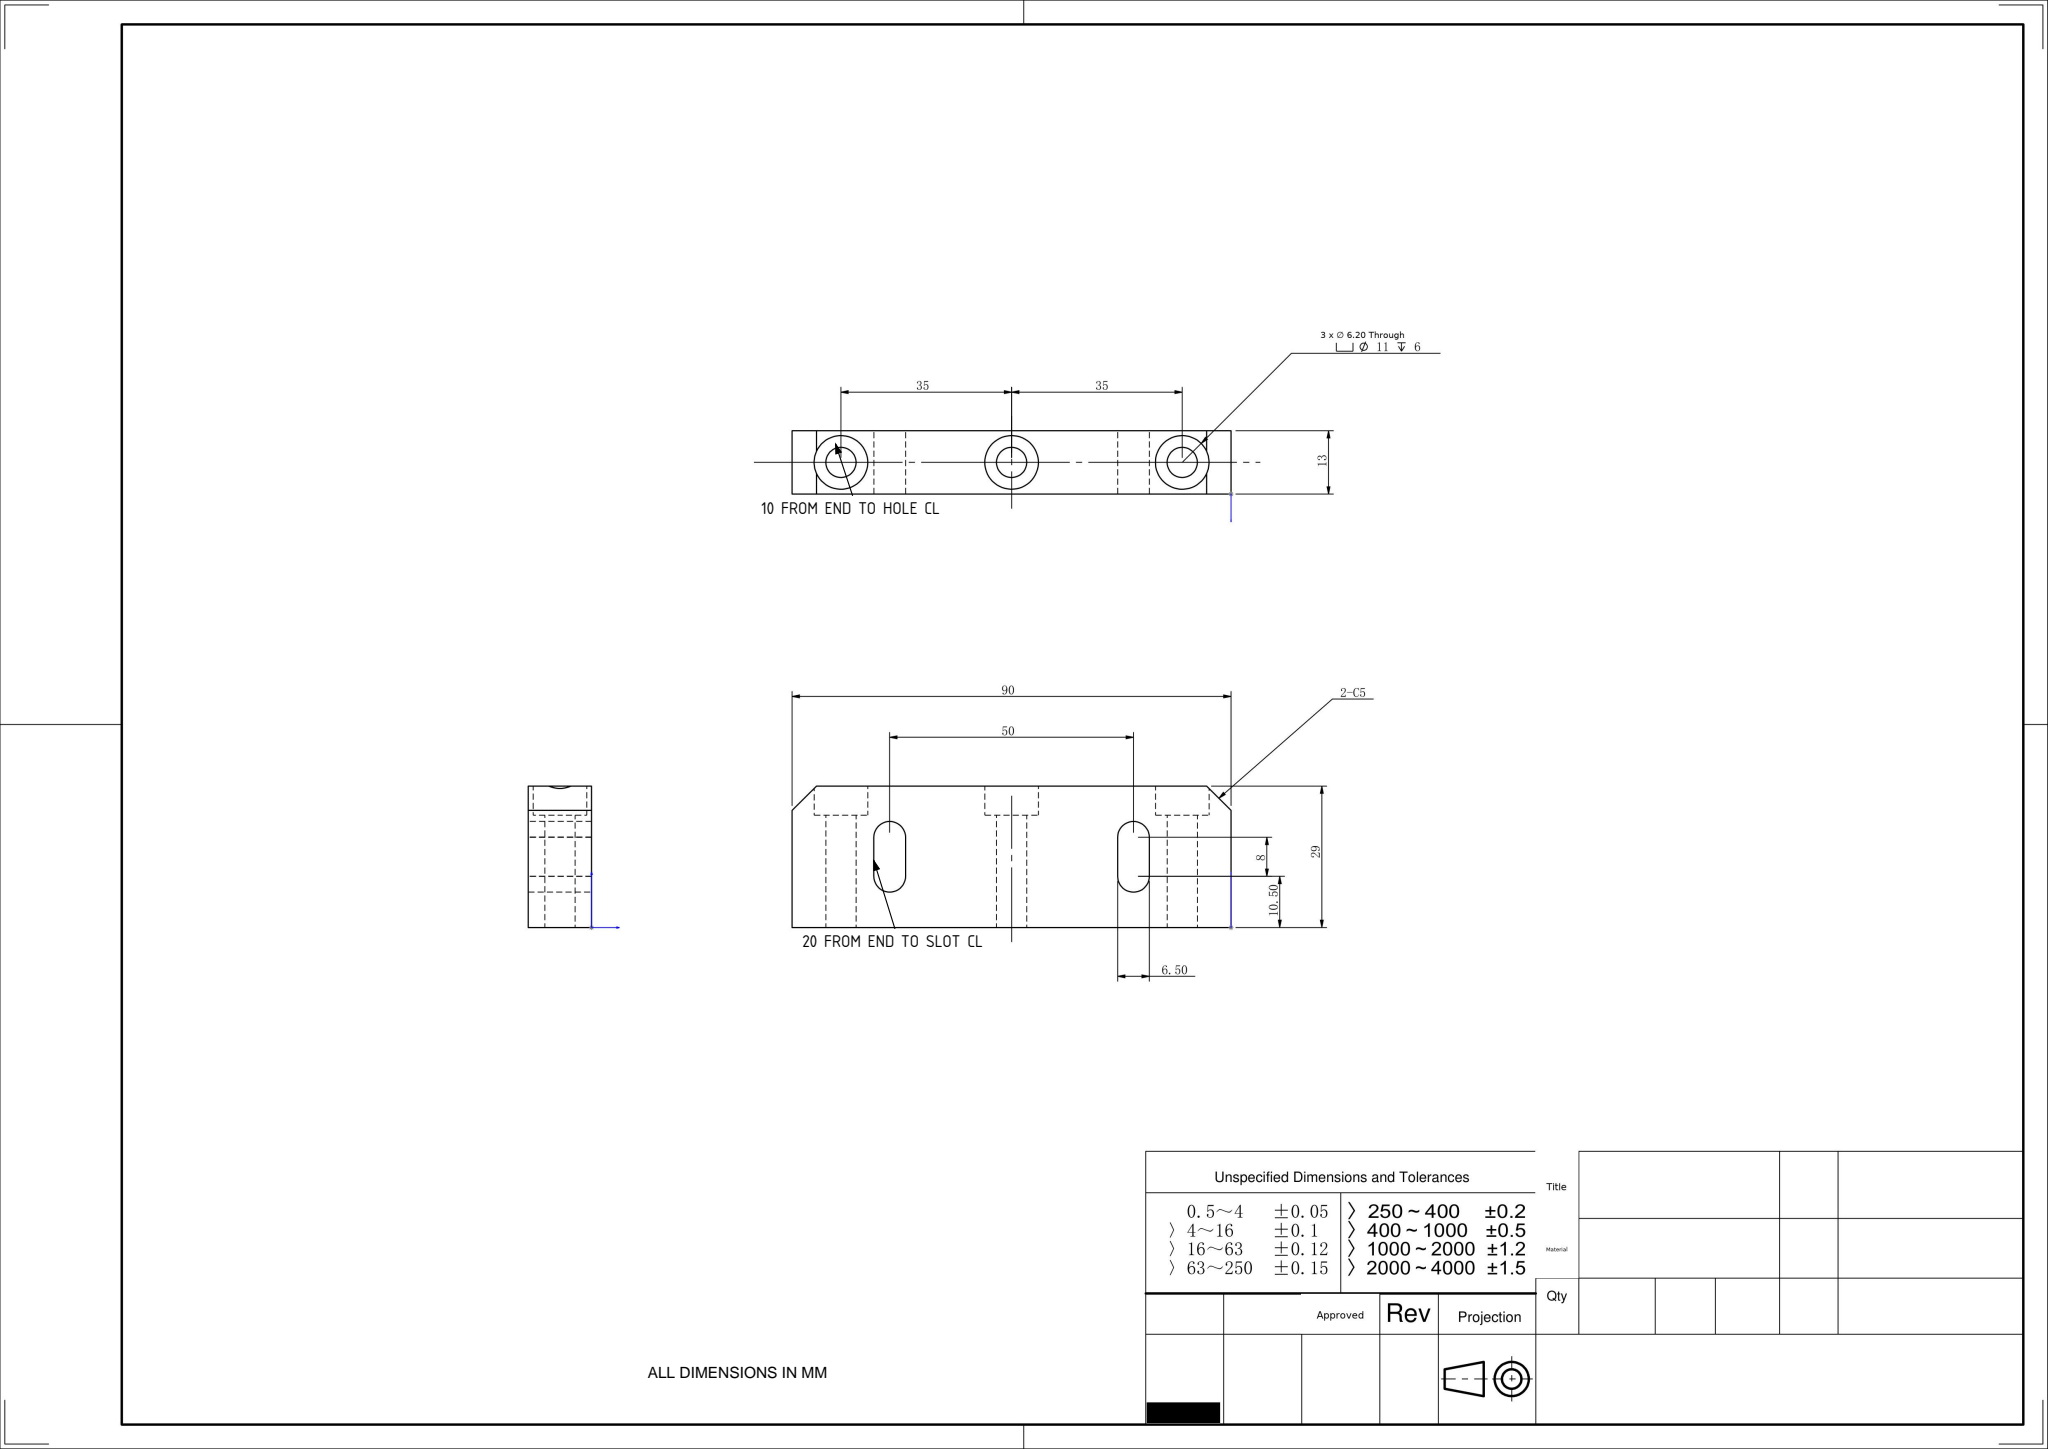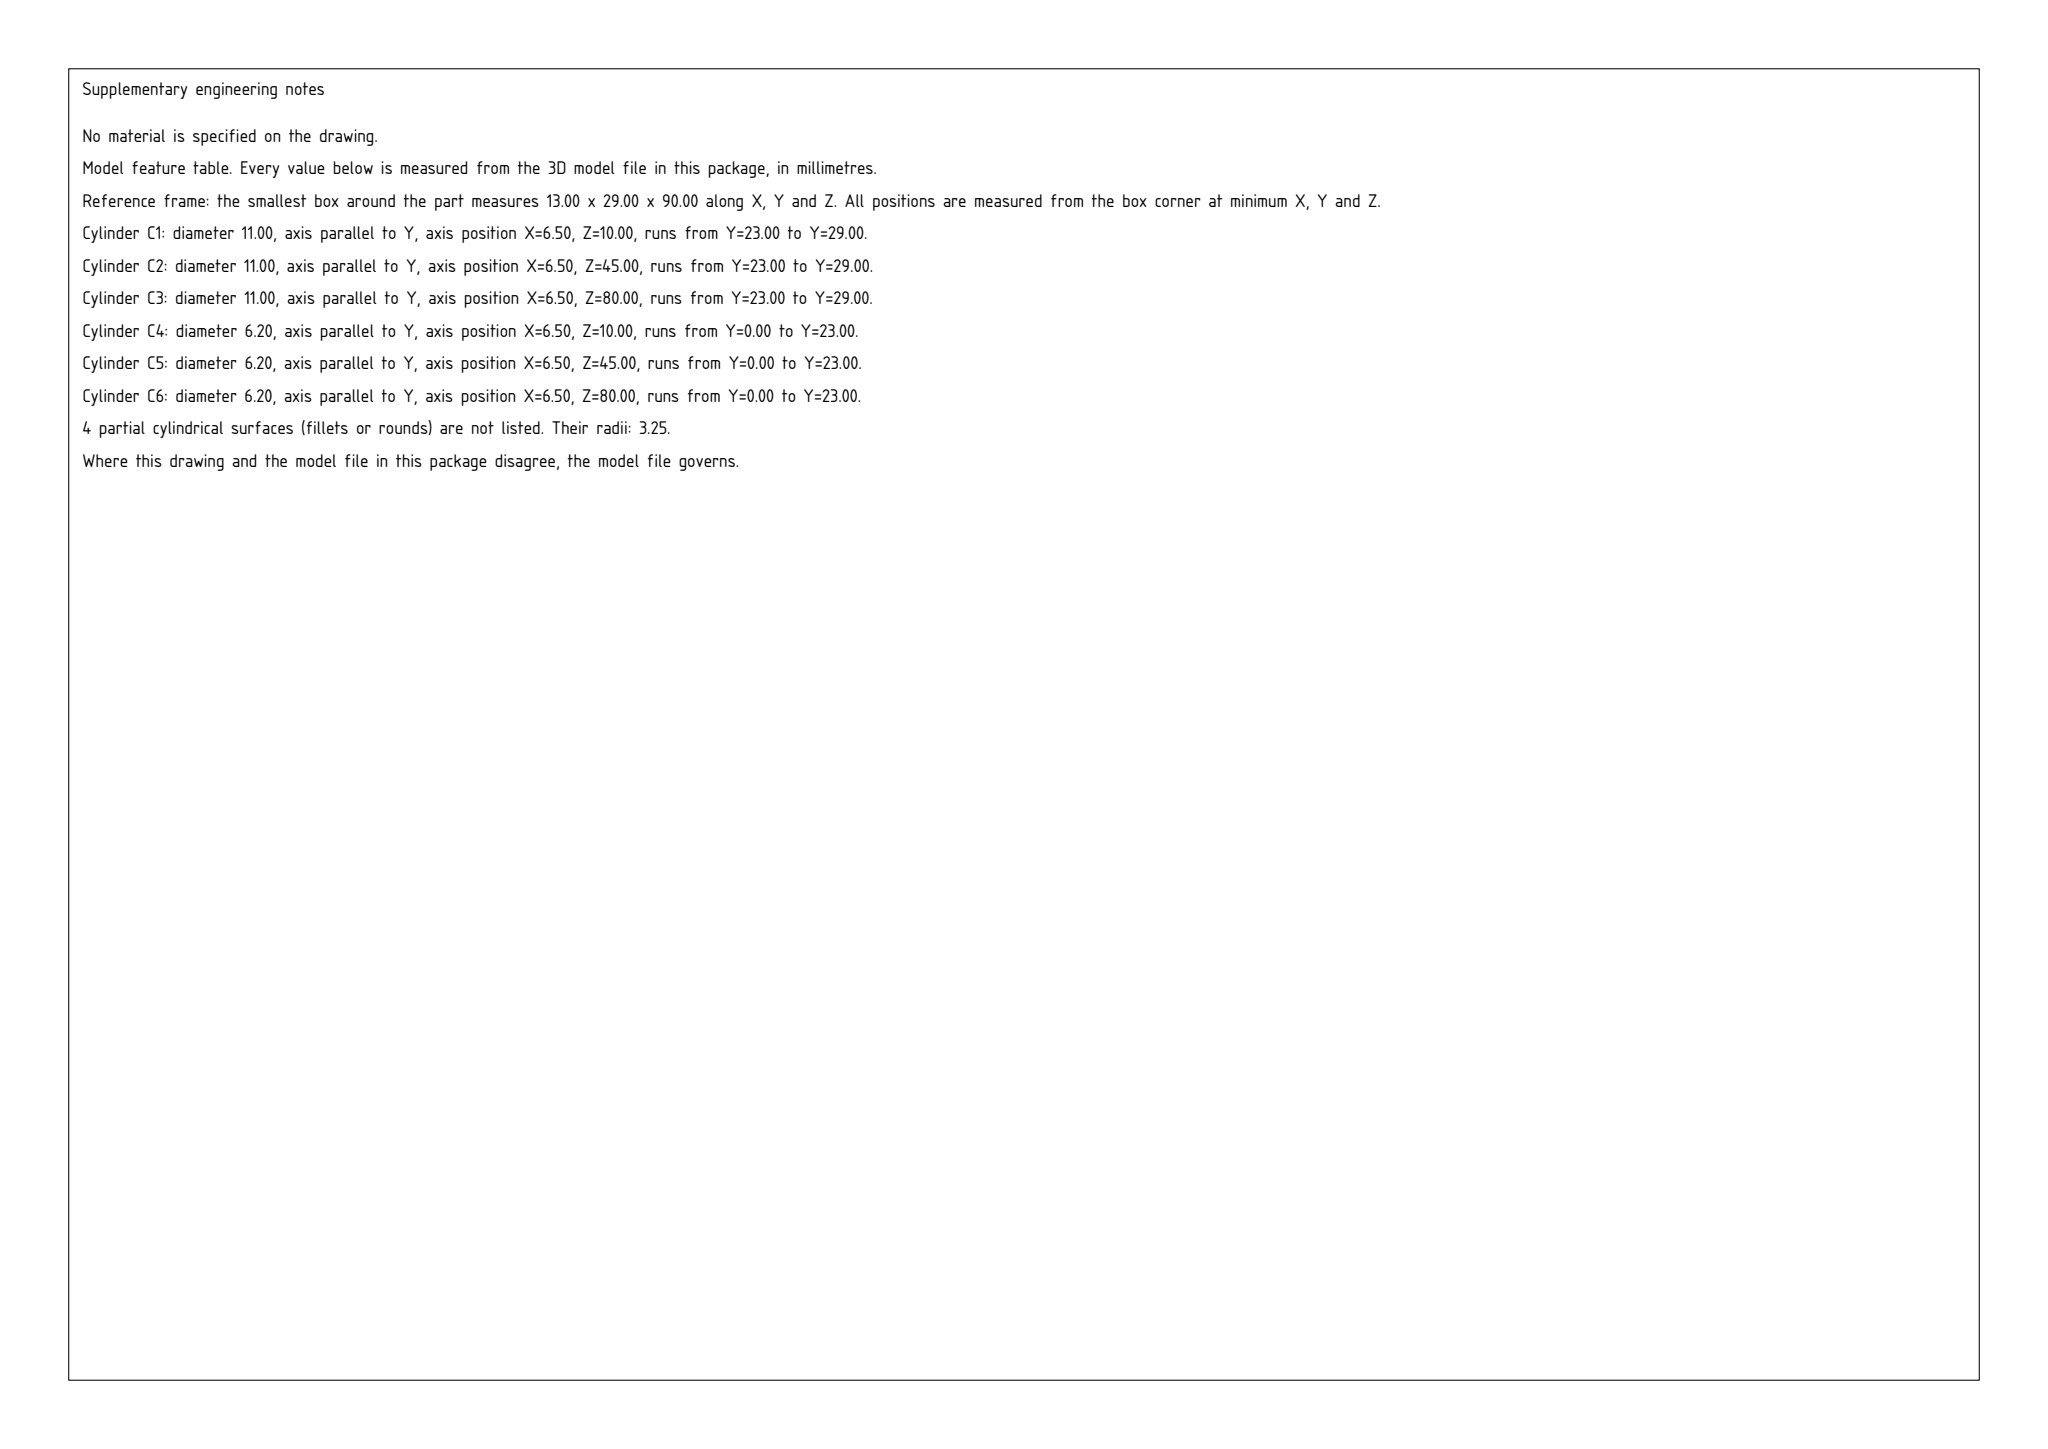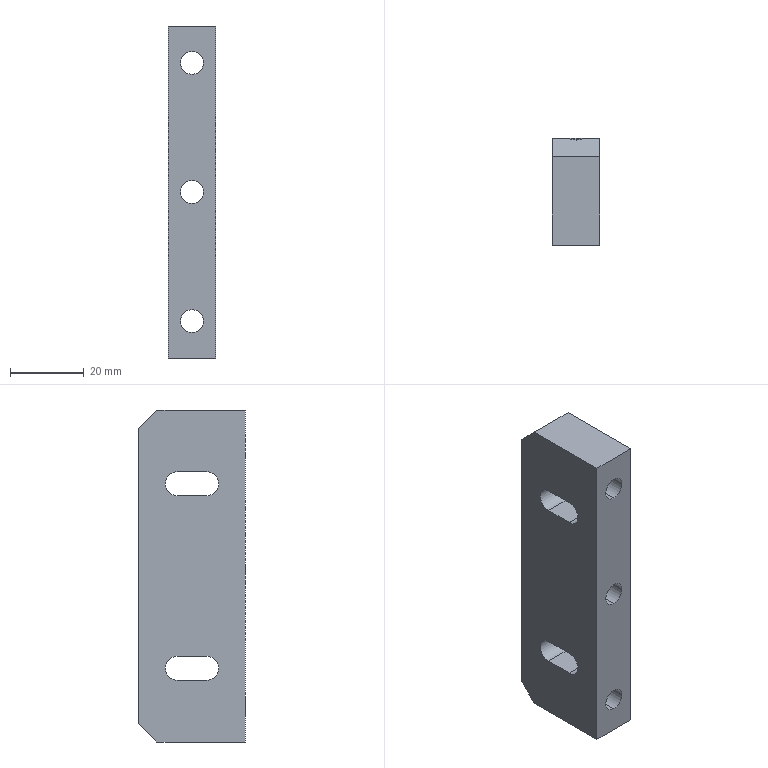Part | SolidWorks | mm | 1 solid | 31 faces | box 13 x 29 x 90 mm | volume 27597 mm3 | cylinder 16 | plane 15 | commonest cylinder face diameters 11 x6 6.2 x6 6.5 x4
Drawing notes:
3 x Ø6.20 C'BORE PATTERN: 10 FROM END TO FIRST HOLE CL | from the solid: Ø6.2/Ø11 holes at z=10, 45, 80; bbox length 90 -> 10 from end, 35 & 35 spacing
2 x 6.50 SLOTS: 20 FROM END TO SLOT CL, 50 CL-CL | from the solid: 6.5 dia slot cylinders at z=20 & 70; bbox length 90 -> 20 from each end